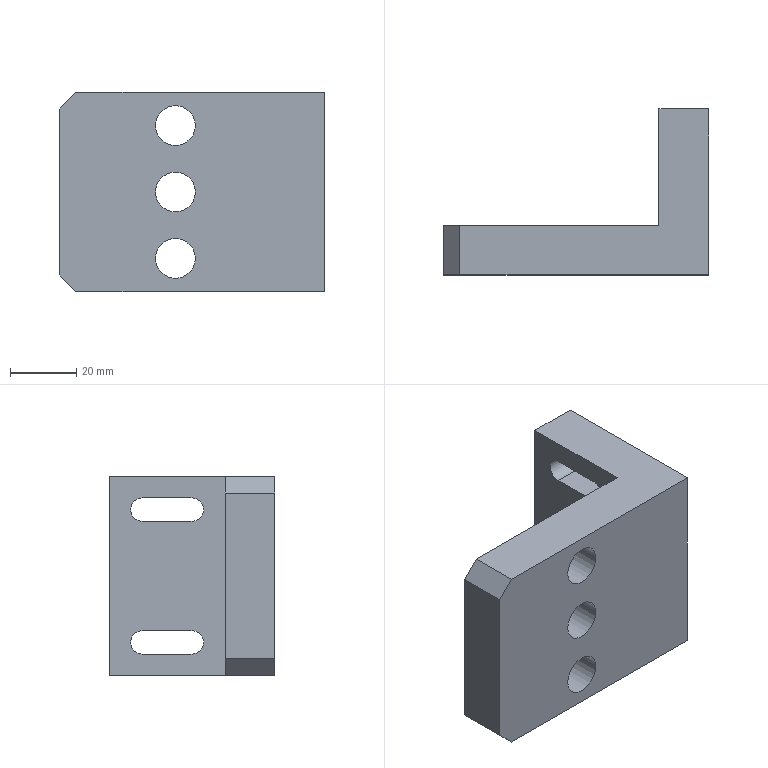Component | SolidWorks | ElectricalBoxAssembly2-1_AuxiliaryWheelAdjustmentSeat-1 | 1 solid | 24 faces | box 80 x 50 x 60 mm | volume 93731 mm3 | plane 14 | cylinder 10 | commonest cylinder face diameters 12 x6 7 x4
build123d program:
from build123d import *

# Parameters (mm, degrees)
BOSS_EXTRUDE1_DEPTH = 30
CUT_EXTRUDE1_DEPTH  = 88.321
SKETCH7_R           = 6
CUT_EXTRUDE2_DEPTH  = 93.331
CHAMFER1_SIZE       = 5


with BuildPart() as part:
    # Sketch1 → Boss-Extrude1 (new, symmetric)
    with BuildSketch(Plane.XY):
        Polygon((0, 0), (0, -50), (80, -50), (80, -35), (15, -35), (15, 0), align=None)
    extrude(amount=BOSS_EXTRUDE1_DEPTH, both=True)

    # Sketch2 → Cut-Extrude1 (cut, through all)
    with BuildSketch(Plane(origin=(15, 0, 0), x_dir=(0, 0, -1), z_dir=(1, 0, 0))):
        with BuildLine():
            Line((-16.5, -10), (-16.5, -25))
            ThreePointArc((-16.5, -25), (-20, -28.5), (-23.5, -25))
            Line((-23.5, -25), (-23.5, -10))
            ThreePointArc((-23.5, -10), (-20, -6.5), (-16.5, -10))
        make_face()
        with BuildLine():
            Line((23.5, -10), (23.5, -25))
            ThreePointArc((23.5, -25), (20, -28.5), (16.5, -25))
            Line((16.5, -25), (16.5, -10))
            ThreePointArc((16.5, -10), (20, -6.5), (23.5, -10))
        make_face()
    extrude(amount=-CUT_EXTRUDE1_DEPTH, mode=Mode.SUBTRACT)

    # Sketch7 → Cut-Extrude2 (cut, through all)
    with BuildSketch(Plane(origin=(0, -35, 0), x_dir=(1, 0, 0), z_dir=(0, 1, 0))):
        with Locations(Location((45, 20, 0), (0, 0, 180))):
            Circle(SKETCH7_R)
        with Locations(Location((45, -20, 0), (0, 0, 180))):
            Circle(SKETCH7_R)
        with Locations(Location((45, 0, 0), (0, 0, 180))):
            Circle(SKETCH7_R)
    extrude(amount=-CUT_EXTRUDE2_DEPTH, mode=Mode.SUBTRACT)

    # Chamfer1
    chamfer1_edges = [part.edges().sort_by_distance(p)[0] for p in [
        (80, -42.5, 30),
        (80, -42.5, -30),
    ]]
    chamfer(chamfer1_edges, length=CHAMFER1_SIZE)


solid = part.part

# Placed as in the assembly
solid = solid.moved(Location((755.468, 489.666, 1526.399), (-180, 0, 180)))
STEP:
#1=CARTESIAN_POINT('',(27.735,17.31,59.307));
#2=VERTEX_POINT('',#1);
#3=CARTESIAN_POINT('',(28.207,17.31,59.307));
#4=VERTEX_POINT('',#3);
#5=CARTESIAN_POINT('',(27.971,17.31,59.307));
#6=DIRECTION('',(-0.,1.,-0.));
#7=DIRECTION('',(1.,0.,0.));
#8=AXIS2_PLACEMENT_3D('',#5,#6,#7);
#9=CIRCLE('',#8,0.2362);
#10=EDGE_CURVE('',#2,#4,#9,.T.);
#11=ORIENTED_EDGE('',*,*,#10,.F.);
#12=CARTESIAN_POINT('',(27.735,17.9,59.307));
#13=VERTEX_POINT('',#12);
#14=CARTESIAN_POINT('',(27.735,17.31,59.307));
#15=DIRECTION('',(-0.,1.,-0.));
#16=VECTOR('',#15,39.37);
#17=LINE('',#14,#16);
#18=EDGE_CURVE('',#2,#13,#17,.T.);
#19=ORIENTED_EDGE('',*,*,#18,.T.);
#20=CARTESIAN_POINT('',(28.207,17.9,59.307));
#21=VERTEX_POINT('',#20);
#22=CARTESIAN_POINT('',(27.971,17.9,59.307));
#23=DIRECTION('',(-0.,1.,-0.));
#24=DIRECTION('',(1.,0.,0.));
#25=AXIS2_PLACEMENT_3D('',#22,#23,#24);
#26=CIRCLE('',#25,0.2362);
#27=EDGE_CURVE('',#13,#21,#26,.T.);
#28=ORIENTED_EDGE('',*,*,#27,.T.);
#29=CARTESIAN_POINT('',(28.207,17.31,59.307));
#30=DIRECTION('',(-0.,1.,-0.));
#31=VECTOR('',#30,39.37);
#32=LINE('',#29,#31);
#33=EDGE_CURVE('',#4,#21,#32,.T.);
#34=ORIENTED_EDGE('',*,*,#33,.F.);
#35=EDGE_LOOP('',(#11,#19,#28,#34));
#36=FACE_OUTER_BOUND('',#35,.T.);
#37=CARTESIAN_POINT('',(27.971,17.31,59.307));
#38=DIRECTION('',(-0.,1.,-0.));
#39=DIRECTION('',(1.,0.,0.));
#40=AXIS2_PLACEMENT_3D('',#37,#38,#39);
#41=CYLINDRICAL_SURFACE('',#40,0.2362);
#42=ADVANCED_FACE('',(#36),#41,.F.);
#43=CARTESIAN_POINT('',(27.735,17.31,60.094));
#44=VERTEX_POINT('',#43);
#45=CARTESIAN_POINT('',(28.207,17.31,60.094));
#46=VERTEX_POINT('',#45);
#47=CARTESIAN_POINT('',(27.971,17.31,60.094));
#48=DIRECTION('',(-0.,1.,-0.));
#49=DIRECTION('',(1.,0.,0.));
#50=AXIS2_PLACEMENT_3D('',#47,#48,#49);
#51=CIRCLE('',#50,0.2362);
#52=EDGE_CURVE('',#44,#46,#51,.T.);
#53=ORIENTED_EDGE('',*,*,#52,.F.);
#54=CARTESIAN_POINT('',(27.735,17.9,60.094));
#55=VERTEX_POINT('',#54);
#56=CARTESIAN_POINT('',(27.735,17.31,60.094));
#57=DIRECTION('',(-0.,1.,-0.));
#58=VECTOR('',#57,39.37);
#59=LINE('',#56,#58);
#60=EDGE_CURVE('',#44,#55,#59,.T.);
#61=ORIENTED_EDGE('',*,*,#60,.T.);
#62=CARTESIAN_POINT('',(28.207,17.9,60.094));
#63=VERTEX_POINT('',#62);
#64=CARTESIAN_POINT('',(27.971,17.9,60.094));
#65=DIRECTION('',(-0.,1.,-0.));
#66=DIRECTION('',(1.,0.,0.));
#67=AXIS2_PLACEMENT_3D('',#64,#65,#66);
#68=CIRCLE('',#67,0.2362);
#69=EDGE_CURVE('',#55,#63,#68,.T.);
#70=ORIENTED_EDGE('',*,*,#69,.T.);
#71=CARTESIAN_POINT('',(28.207,17.31,60.094));
#72=DIRECTION('',(-0.,1.,-0.));
#73=VECTOR('',#72,39.37);
#74=LINE('',#71,#73);
#75=EDGE_CURVE('',#46,#63,#74,.T.);
#76=ORIENTED_EDGE('',*,*,#75,.F.);
#77=EDGE_LOOP('',(#53,#61,#70,#76));
#78=FACE_OUTER_BOUND('',#77,.T.);
#79=CARTESIAN_POINT('',(27.971,17.31,60.094));
#80=DIRECTION('',(-0.,1.,-0.));
#81=DIRECTION('',(1.,0.,0.));
#82=AXIS2_PLACEMENT_3D('',#79,#80,#81);
#83=CYLINDRICAL_SURFACE('',#82,0.2362);
#84=ADVANCED_FACE('',(#78),#83,.F.);
#85=CARTESIAN_POINT('',(27.735,17.31,60.882));
#86=VERTEX_POINT('',#85);
#87=CARTESIAN_POINT('',(28.207,17.31,60.882));
#88=VERTEX_POINT('',#87);
#89=CARTESIAN_POINT('',(27.971,17.31,60.882));
#90=DIRECTION('',(-0.,1.,-0.));
#91=DIRECTION('',(1.,0.,0.));
#92=AXIS2_PLACEMENT_3D('',#89,#90,#91);
#93=CIRCLE('',#92,0.2362);
#94=EDGE_CURVE('',#86,#88,#93,.T.);
#95=ORIENTED_EDGE('',*,*,#94,.F.);
#96=CARTESIAN_POINT('',(27.735,17.9,60.882));
#97=VERTEX_POINT('',#96);
#98=CARTESIAN_POINT('',(27.735,17.31,60.882));
#99=DIRECTION('',(-0.,1.,-0.));
#100=VECTOR('',#99,39.37);
#101=LINE('',#98,#100);
#102=EDGE_CURVE('',#86,#97,#101,.T.);
#103=ORIENTED_EDGE('',*,*,#102,.T.);
#104=CARTESIAN_POINT('',(28.207,17.9,60.882));
#105=VERTEX_POINT('',#104);
#106=CARTESIAN_POINT('',(27.971,17.9,60.882));
#107=DIRECTION('',(-0.,1.,-0.));
#108=DIRECTION('',(1.,0.,0.));
#109=AXIS2_PLACEMENT_3D('',#106,#107,#108);
#110=CIRCLE('',#109,0.2362);
#111=EDGE_CURVE('',#97,#105,#110,.T.);
#112=ORIENTED_EDGE('',*,*,#111,.T.);
#113=CARTESIAN_POINT('',(28.207,17.31,60.882));
#114=DIRECTION('',(-0.,1.,-0.));
#115=VECTOR('',#114,39.37);
#116=LINE('',#113,#115);
#117=EDGE_CURVE('',#88,#105,#116,.T.);
#118=ORIENTED_EDGE('',*,*,#117,.F.);
#119=EDGE_LOOP('',(#95,#103,#112,#118));
#120=FACE_OUTER_BOUND('',#119,.T.);
#121=CARTESIAN_POINT('',(27.971,17.31,60.882));
#122=DIRECTION('',(-0.,1.,-0.));
#123=DIRECTION('',(1.,0.,0.));
#124=AXIS2_PLACEMENT_3D('',#121,#122,#123);
#125=CYLINDRICAL_SURFACE('',#124,0.2362);
#126=ADVANCED_FACE('',(#120),#125,.F.);
#127=CARTESIAN_POINT('',(29.152,19.278,61.276));
#128=VERTEX_POINT('',#127);
#129=CARTESIAN_POINT('',(29.743,19.278,61.276));
#130=VERTEX_POINT('',#129);
#131=CARTESIAN_POINT('',(29.152,19.278,61.276));
#132=DIRECTION('',(1.,0.,0.));
#133=VECTOR('',#132,39.37);
#134=LINE('',#131,#133);
#135=EDGE_CURVE('',#128,#130,#134,.T.);
#136=ORIENTED_EDGE('',*,*,#135,.T.);
#137=CARTESIAN_POINT('',(29.743,19.278,58.913));
#138=VERTEX_POINT('',#137);
#139=CARTESIAN_POINT('',(29.743,19.278,58.913));
#140=DIRECTION('',(-0.,0.,1.));
#141=VECTOR('',#140,39.37);
#142=LINE('',#139,#141);
#143=EDGE_CURVE('',#138,#130,#142,.T.);
#144=ORIENTED_EDGE('',*,*,#143,.F.);
#145=CARTESIAN_POINT('',(29.152,19.278,58.913));
#146=VERTEX_POINT('',#145);
#147=CARTESIAN_POINT('',(29.152,19.278,58.913));
#148=DIRECTION('',(1.,0.,0.));
#149=VECTOR('',#148,39.37);
#150=LINE('',#147,#149);
#151=EDGE_CURVE('',#146,#138,#150,.T.);
#152=ORIENTED_EDGE('',*,*,#151,.F.);
#153=CARTESIAN_POINT('',(29.152,19.278,58.913));
#154=DIRECTION('',(-0.,0.,1.));
#155=VECTOR('',#154,39.37);
#156=LINE('',#153,#155);
#157=EDGE_CURVE('',#146,#128,#156,.T.);
#158=ORIENTED_EDGE('',*,*,#157,.T.);
#159=EDGE_LOOP('',(#136,#144,#152,#158));
#160=FACE_OUTER_BOUND('',#159,.T.);
#161=CARTESIAN_POINT('',(29.152,19.278,58.913));
#162=DIRECTION('',(0.,-1.,0.));
#163=DIRECTION('',(-1.,-0.,-0.));
#164=AXIS2_PLACEMENT_3D('',#161,#162,#163);
#165=PLANE('',#164);
#166=ADVANCED_FACE('',(#160),#165,.F.);
#167=CARTESIAN_POINT('',(29.743,18.294,61.02));
#168=VERTEX_POINT('',#167);
#169=CARTESIAN_POINT('',(29.743,18.884,61.02));
#170=VERTEX_POINT('',#169);
#171=CARTESIAN_POINT('',(29.743,18.884,61.02));
#172=DIRECTION('',(-0.,1.,-0.));
#173=VECTOR('',#172,39.37);
#174=LINE('',#171,#173);
#175=EDGE_CURVE('',#168,#170,#174,.T.);
#176=ORIENTED_EDGE('',*,*,#175,.T.);
#177=CARTESIAN_POINT('',(29.743,18.884,60.744));
#178=VERTEX_POINT('',#177);
#179=CARTESIAN_POINT('',(29.743,18.884,60.882));
#180=DIRECTION('',(-1.,-0.,-0.));
#181=DIRECTION('',(0.,0.,1.));
#182=AXIS2_PLACEMENT_3D('',#179,#180,#181);
#183=CIRCLE('',#182,0.1378);
#184=EDGE_CURVE('',#170,#178,#183,.T.);
#185=ORIENTED_EDGE('',*,*,#184,.T.);
#186=CARTESIAN_POINT('',(29.743,18.294,60.744));
#187=VERTEX_POINT('',#186);
#188=CARTESIAN_POINT('',(29.743,18.884,60.744));
#189=DIRECTION('',(0.,-1.,0.));
#190=VECTOR('',#189,39.37);
#191=LINE('',#188,#190);
#192=EDGE_CURVE('',#178,#187,#191,.T.);
#193=ORIENTED_EDGE('',*,*,#192,.T.);
#194=CARTESIAN_POINT('',(29.743,18.294,60.882));
#195=DIRECTION('',(-1.,-0.,-0.));
#196=DIRECTION('',(0.,0.,1.));
#197=AXIS2_PLACEMENT_3D('',#194,#195,#196);
#198=CIRCLE('',#197,0.1378);
#199=EDGE_CURVE('',#187,#168,#198,.T.);
#200=ORIENTED_EDGE('',*,*,#199,.T.);
#201=EDGE_LOOP('',(#176,#185,#193,#200));
#202=FACE_BOUND('',#201,.T.);
#203=CARTESIAN_POINT('',(29.743,18.294,59.445));
#204=VERTEX_POINT('',#203);
#205=CARTESIAN_POINT('',(29.743,18.884,59.445));
#206=VERTEX_POINT('',#205);
#207=CARTESIAN_POINT('',(29.743,18.884,59.445));
#208=DIRECTION('',(-0.,1.,-0.));
#209=VECTOR('',#208,39.37);
#210=LINE('',#207,#209);
#211=EDGE_CURVE('',#204,#206,#210,.T.);
#212=ORIENTED_EDGE('',*,*,#211,.T.);
#213=CARTESIAN_POINT('',(29.743,18.884,59.169));
#214=VERTEX_POINT('',#213);
#215=CARTESIAN_POINT('',(29.743,18.884,59.307));
#216=DIRECTION('',(-1.,-0.,-0.));
#217=DIRECTION('',(0.,0.,1.));
#218=AXIS2_PLACEMENT_3D('',#215,#216,#217);
#219=CIRCLE('',#218,0.1378);
#220=EDGE_CURVE('',#206,#214,#219,.T.);
#221=ORIENTED_EDGE('',*,*,#220,.T.);
#222=CARTESIAN_POINT('',(29.743,18.294,59.169));
#223=VERTEX_POINT('',#222);
#224=CARTESIAN_POINT('',(29.743,18.884,59.169));
#225=DIRECTION('',(0.,-1.,0.));
#226=VECTOR('',#225,39.37);
#227=LINE('',#224,#226);
#228=EDGE_CURVE('',#214,#223,#227,.T.);
#229=ORIENTED_EDGE('',*,*,#228,.T.);
#230=CARTESIAN_POINT('',(29.743,18.294,59.307));
#231=DIRECTION('',(-1.,-0.,-0.));
#232=DIRECTION('',(0.,0.,1.));
#233=AXIS2_PLACEMENT_3D('',#230,#231,#232);
#234=CIRCLE('',#233,0.1378);
#235=EDGE_CURVE('',#223,#204,#234,.T.);
#236=ORIENTED_EDGE('',*,*,#235,.T.);
#237=EDGE_LOOP('',(#212,#221,#229,#236));
#238=FACE_BOUND('',#237,.T.);
#239=CARTESIAN_POINT('',(29.743,17.31,61.276));
#240=VERTEX_POINT('',#239);
#241=CARTESIAN_POINT('',(29.743,19.278,61.276));
#242=DIRECTION('',(0.,-1.,0.));
#243=VECTOR('',#242,39.37);
#244=LINE('',#241,#243);
#245=EDGE_CURVE('',#130,#240,#244,.T.);
#246=ORIENTED_EDGE('',*,*,#245,.T.);
#247=CARTESIAN_POINT('',(29.743,17.31,58.913));
#248=VERTEX_POINT('',#247);
#249=CARTESIAN_POINT('',(29.743,17.31,58.913));
#250=DIRECTION('',(-0.,0.,1.));
#251=VECTOR('',#250,39.37);
#252=LINE('',#249,#251);
#253=EDGE_CURVE('',#248,#240,#252,.T.);
#254=ORIENTED_EDGE('',*,*,#253,.F.);
#255=CARTESIAN_POINT('',(29.743,19.278,58.913));
#256=DIRECTION('',(0.,-1.,0.));
#257=VECTOR('',#256,39.37);
#258=LINE('',#255,#257);
#259=EDGE_CURVE('',#138,#248,#258,.T.);
#260=ORIENTED_EDGE('',*,*,#259,.F.);
#261=ORIENTED_EDGE('',*,*,#143,.T.);
#262=EDGE_LOOP('',(#246,#254,#260,#261));
#263=FACE_OUTER_BOUND('',#262,.T.);
#264=CARTESIAN_POINT('',(29.743,19.278,58.913));
#265=DIRECTION('',(-1.,-0.,-0.));
#266=DIRECTION('',(-0.,1.,-0.));
#267=AXIS2_PLACEMENT_3D('',#264,#265,#266);
#268=PLANE('',#267);
#269=ADVANCED_FACE('',(#202,#238,#263),#268,.F.);
#270=CARTESIAN_POINT('',(27.971,17.31,59.307));
#271=DIRECTION('',(-0.,1.,-0.));
#272=DIRECTION('',(1.,0.,0.));
#273=AXIS2_PLACEMENT_3D('',#270,#271,#272);
#274=CIRCLE('',#273,0.2362);
#275=EDGE_CURVE('',#4,#2,#274,.T.);
#276=ORIENTED_EDGE('',*,*,#275,.T.);
#277=ORIENTED_EDGE('',*,*,#10,.T.);
#278=EDGE_LOOP('',(#276,#277));
#279=FACE_BOUND('',#278,.T.);
#280=CARTESIAN_POINT('',(27.971,17.31,60.094));
#281=DIRECTION('',(-0.,1.,-0.));
#282=DIRECTION('',(1.,0.,0.));
#283=AXIS2_PLACEMENT_3D('',#280,#281,#282);
#284=CIRCLE('',#283,0.2362);
#285=EDGE_CURVE('',#46,#44,#284,.T.);
#286=ORIENTED_EDGE('',*,*,#285,.T.);
#287=ORIENTED_EDGE('',*,*,#52,.T.);
#288=EDGE_LOOP('',(#286,#287));
#289=FACE_BOUND('',#288,.T.);
#290=CARTESIAN_POINT('',(27.971,17.31,60.882));
#291=DIRECTION('',(-0.,1.,-0.));
#292=DIRECTION('',(1.,0.,0.));
#293=AXIS2_PLACEMENT_3D('',#290,#291,#292);
#294=CIRCLE('',#293,0.2362);
#295=EDGE_CURVE('',#88,#86,#294,.T.);
#296=ORIENTED_EDGE('',*,*,#295,.T.);
#297=ORIENTED_EDGE('',*,*,#94,.T.);
#298=EDGE_LOOP('',(#296,#297));
#299=FACE_BOUND('',#298,.T.);
#300=CARTESIAN_POINT('',(26.593,17.31,59.11));
#301=VERTEX_POINT('',#300);
#302=CARTESIAN_POINT('',(26.593,17.31,61.079));
#303=VERTEX_POINT('',#302);
#304=CARTESIAN_POINT('',(26.593,17.31,58.913));
#305=DIRECTION('',(-0.,0.,1.));
#306=VECTOR('',#305,39.37);
#307=LINE('',#304,#306);
#308=EDGE_CURVE('',#301,#303,#307,.T.);
#309=ORIENTED_EDGE('',*,*,#308,.F.);
#310=CARTESIAN_POINT('',(26.79,17.31,58.913));
#311=VERTEX_POINT('',#310);
#312=CARTESIAN_POINT('',(26.79,17.31,58.913));
#313=DIRECTION('',(0.7071,0.,-0.7071));
#314=VECTOR('',#313,39.37);
#315=LINE('',#312,#314);
#316=EDGE_CURVE('',#301,#311,#315,.T.);
#317=ORIENTED_EDGE('',*,*,#316,.T.);
#318=CARTESIAN_POINT('',(29.743,17.31,58.913));
#319=DIRECTION('',(-1.,-0.,-0.));
#320=VECTOR('',#319,39.37);
#321=LINE('',#318,#320);
#322=EDGE_CURVE('',#248,#311,#321,.T.);
#323=ORIENTED_EDGE('',*,*,#322,.F.);
#324=ORIENTED_EDGE('',*,*,#253,.T.);
#325=CARTESIAN_POINT('',(26.79,17.31,61.276));
#326=VERTEX_POINT('',#325);
#327=CARTESIAN_POINT('',(29.743,17.31,61.276));
#328=DIRECTION('',(-1.,-0.,-0.));
#329=VECTOR('',#328,39.37);
#330=LINE('',#327,#329);
#331=EDGE_CURVE('',#240,#326,#330,.T.);
#332=ORIENTED_EDGE('',*,*,#331,.T.);
#333=CARTESIAN_POINT('',(26.593,17.31,61.079));
#334=DIRECTION('',(-0.7071,-0.,-0.7071));
#335=VECTOR('',#334,39.37);
#336=LINE('',#333,#335);
#337=EDGE_CURVE('',#326,#303,#336,.T.);
#338=ORIENTED_EDGE('',*,*,#337,.T.);
#339=EDGE_LOOP('',(#309,#317,#323,#324,#332,#338));
#340=FACE_OUTER_BOUND('',#339,.T.);
#341=CARTESIAN_POINT('',(29.743,17.31,58.913));
#342=DIRECTION('',(-0.,1.,-0.));
#343=DIRECTION('',(0.,-0.,-1.));
#344=AXIS2_PLACEMENT_3D('',#341,#342,#343);
#345=PLANE('',#344);
#346=ADVANCED_FACE('',(#279,#289,#299,#340),#345,.F.);
#347=CARTESIAN_POINT('',(26.593,17.9,59.11));
#348=VERTEX_POINT('',#347);
#349=CARTESIAN_POINT('',(26.593,17.9,61.079));
#350=VERTEX_POINT('',#349);
#351=CARTESIAN_POINT('',(26.593,17.9,58.913));
#352=DIRECTION('',(-0.,0.,1.));
#353=VECTOR('',#352,39.37);
#354=LINE('',#351,#353);
#355=EDGE_CURVE('',#348,#350,#354,.T.);
#356=ORIENTED_EDGE('',*,*,#355,.F.);
#357=CARTESIAN_POINT('',(26.593,17.31,59.11));
#358=DIRECTION('',(0.,-1.,0.));
#359=VECTOR('',#358,39.37);
#360=LINE('',#357,#359);
#361=EDGE_CURVE('',#348,#301,#360,.T.);
#362=ORIENTED_EDGE('',*,*,#361,.T.);
#363=ORIENTED_EDGE('',*,*,#308,.T.);
#364=CARTESIAN_POINT('',(26.593,17.31,61.079));
#365=DIRECTION('',(-0.,1.,-0.));
#366=VECTOR('',#365,39.37);
#367=LINE('',#364,#366);
#368=EDGE_CURVE('',#303,#350,#367,.T.);
#369=ORIENTED_EDGE('',*,*,#368,.T.);
#370=EDGE_LOOP('',(#356,#362,#363,#369));
#371=FACE_OUTER_BOUND('',#370,.T.);
#372=CARTESIAN_POINT('',(26.593,17.31,58.913));
#373=DIRECTION('',(1.,0.,0.));
#374=DIRECTION('',(0.,-0.,-1.));
#375=AXIS2_PLACEMENT_3D('',#372,#373,#374);
#376=PLANE('',#375);
#377=ADVANCED_FACE('',(#371),#376,.F.);
#378=CARTESIAN_POINT('',(27.971,17.9,59.307));
#379=DIRECTION('',(-0.,1.,-0.));
#380=DIRECTION('',(1.,0.,0.));
#381=AXIS2_PLACEMENT_3D('',#378,#379,#380);
#382=CIRCLE('',#381,0.2362);
#383=EDGE_CURVE('',#21,#13,#382,.T.);
#384=ORIENTED_EDGE('',*,*,#383,.F.);
#385=ORIENTED_EDGE('',*,*,#27,.F.);
#386=EDGE_LOOP('',(#384,#385));
#387=FACE_BOUND('',#386,.T.);
#388=CARTESIAN_POINT('',(27.971,17.9,60.094));
#389=DIRECTION('',(-0.,1.,-0.));
#390=DIRECTION('',(1.,0.,0.));
#391=AXIS2_PLACEMENT_3D('',#388,#389,#390);
#392=CIRCLE('',#391,0.2362);
#393=EDGE_CURVE('',#63,#55,#392,.T.);
#394=ORIENTED_EDGE('',*,*,#393,.F.);
#395=ORIENTED_EDGE('',*,*,#69,.F.);
#396=EDGE_LOOP('',(#394,#395));
#397=FACE_BOUND('',#396,.T.);
#398=CARTESIAN_POINT('',(27.971,17.9,60.882));
#399=DIRECTION('',(-0.,1.,-0.));
#400=DIRECTION('',(1.,0.,0.));
#401=AXIS2_PLACEMENT_3D('',#398,#399,#400);
#402=CIRCLE('',#401,0.2362);
#403=EDGE_CURVE('',#105,#97,#402,.T.);
#404=ORIENTED_EDGE('',*,*,#403,.F.);
#405=ORIENTED_EDGE('',*,*,#111,.F.);
#406=EDGE_LOOP('',(#404,#405));
#407=FACE_BOUND('',#406,.T.);
#408=CARTESIAN_POINT('',(26.79,17.9,58.913));
#409=VERTEX_POINT('',#408);
#410=CARTESIAN_POINT('',(29.152,17.9,58.913));
#411=VERTEX_POINT('',#410);
#412=CARTESIAN_POINT('',(26.593,17.9,58.913));
#413=DIRECTION('',(1.,0.,0.));
#414=VECTOR('',#413,39.37);
#415=LINE('',#412,#414);
#416=EDGE_CURVE('',#409,#411,#415,.T.);
#417=ORIENTED_EDGE('',*,*,#416,.F.);
#418=CARTESIAN_POINT('',(26.79,17.9,58.913));
#419=DIRECTION('',(-0.7071,-0.,0.7071));
#420=VECTOR('',#419,39.37);
#421=LINE('',#418,#420);
#422=EDGE_CURVE('',#409,#348,#421,.T.);
#423=ORIENTED_EDGE('',*,*,#422,.T.);
#424=ORIENTED_EDGE('',*,*,#355,.T.);
#425=CARTESIAN_POINT('',(26.79,17.9,61.276));
#426=VERTEX_POINT('',#425);
#427=CARTESIAN_POINT('',(26.593,17.9,61.079));
#428=DIRECTION('',(0.7071,0.,0.7071));
#429=VECTOR('',#428,39.37);
#430=LINE('',#427,#429);
#431=EDGE_CURVE('',#350,#426,#430,.T.);
#432=ORIENTED_EDGE('',*,*,#431,.T.);
#433=CARTESIAN_POINT('',(29.152,17.9,61.276));
#434=VERTEX_POINT('',#433);
#435=CARTESIAN_POINT('',(26.593,17.9,61.276));
#436=DIRECTION('',(1.,0.,0.));
#437=VECTOR('',#436,39.37);
#438=LINE('',#435,#437);
#439=EDGE_CURVE('',#426,#434,#438,.T.);
#440=ORIENTED_EDGE('',*,*,#439,.T.);
#441=CARTESIAN_POINT('',(29.152,17.9,58.913));
#442=DIRECTION('',(-0.,0.,1.));
#443=VECTOR('',#442,39.37);
#444=LINE('',#441,#443);
#445=EDGE_CURVE('',#411,#434,#444,.T.);
#446=ORIENTED_EDGE('',*,*,#445,.F.);
#447=EDGE_LOOP('',(#417,#423,#424,#432,#440,#446));
#448=FACE_OUTER_BOUND('',#447,.T.);
#449=CARTESIAN_POINT('',(26.593,17.9,58.913));
#450=DIRECTION('',(0.,-1.,0.));
#451=DIRECTION('',(-1.,-0.,-0.));
#452=AXIS2_PLACEMENT_3D('',#449,#450,#451);
#453=PLANE('',#452);
#454=ADVANCED_FACE('',(#387,#397,#407,#448),#453,.F.);
#455=CARTESIAN_POINT('',(29.152,18.884,60.744));
#456=VERTEX_POINT('',#455);
#457=CARTESIAN_POINT('',(29.152,18.294,60.744));
#458=VERTEX_POINT('',#457);
#459=CARTESIAN_POINT('',(29.152,18.884,60.744));
#460=DIRECTION('',(0.,-1.,0.));
#461=VECTOR('',#460,39.37);
#462=LINE('',#459,#461);
#463=EDGE_CURVE('',#456,#458,#462,.T.);
#464=ORIENTED_EDGE('',*,*,#463,.F.);
#465=CARTESIAN_POINT('',(29.152,18.884,61.02));
#466=VERTEX_POINT('',#465);
#467=CARTESIAN_POINT('',(29.152,18.884,60.882));
#468=DIRECTION('',(-1.,-0.,-0.));
#469=DIRECTION('',(0.,0.,1.));
#470=AXIS2_PLACEMENT_3D('',#467,#468,#469);
#471=CIRCLE('',#470,0.1378);
#472=EDGE_CURVE('',#466,#456,#471,.T.);
#473=ORIENTED_EDGE('',*,*,#472,.F.);
#474=CARTESIAN_POINT('',(29.152,18.294,61.02));
#475=VERTEX_POINT('',#474);
#476=CARTESIAN_POINT('',(29.152,18.884,61.02));
#477=DIRECTION('',(-0.,1.,-0.));
#478=VECTOR('',#477,39.37);
#479=LINE('',#476,#478);
#480=EDGE_CURVE('',#475,#466,#479,.T.);
#481=ORIENTED_EDGE('',*,*,#480,.F.);
#482=CARTESIAN_POINT('',(29.152,18.294,60.882));
#483=DIRECTION('',(-1.,-0.,-0.));
#484=DIRECTION('',(0.,0.,1.));
#485=AXIS2_PLACEMENT_3D('',#482,#483,#484);
#486=CIRCLE('',#485,0.1378);
#487=EDGE_CURVE('',#458,#475,#486,.T.);
#488=ORIENTED_EDGE('',*,*,#487,.F.);
#489=EDGE_LOOP('',(#464,#473,#481,#488));
#490=FACE_BOUND('',#489,.T.);
#491=CARTESIAN_POINT('',(29.152,18.884,59.169));
#492=VERTEX_POINT('',#491);
#493=CARTESIAN_POINT('',(29.152,18.294,59.169));
#494=VERTEX_POINT('',#493);
#495=CARTESIAN_POINT('',(29.152,18.884,59.169));
#496=DIRECTION('',(0.,-1.,0.));
#497=VECTOR('',#496,39.37);
#498=LINE('',#495,#497);
#499=EDGE_CURVE('',#492,#494,#498,.T.);
#500=ORIENTED_EDGE('',*,*,#499,.F.);
#501=CARTESIAN_POINT('',(29.152,18.884,59.445));
#502=VERTEX_POINT('',#501);
#503=CARTESIAN_POINT('',(29.152,18.884,59.307));
#504=DIRECTION('',(-1.,-0.,-0.));
#505=DIRECTION('',(0.,0.,1.));
#506=AXIS2_PLACEMENT_3D('',#503,#504,#505);
#507=CIRCLE('',#506,0.1378);
#508=EDGE_CURVE('',#502,#492,#507,.T.);
#509=ORIENTED_EDGE('',*,*,#508,.F.);
#510=CARTESIAN_POINT('',(29.152,18.294,59.445));
#511=VERTEX_POINT('',#510);
#512=CARTESIAN_POINT('',(29.152,18.884,59.445));
#513=DIRECTION('',(-0.,1.,-0.));
#514=VECTOR('',#513,39.37);
#515=LINE('',#512,#514);
#516=EDGE_CURVE('',#511,#502,#515,.T.);
#517=ORIENTED_EDGE('',*,*,#516,.F.);
#518=CARTESIAN_POINT('',(29.152,18.294,59.307));
#519=DIRECTION('',(-1.,-0.,-0.));
#520=DIRECTION('',(0.,0.,1.));
#521=AXIS2_PLACEMENT_3D('',#518,#519,#520);
#522=CIRCLE('',#521,0.1378);
#523=EDGE_CURVE('',#494,#511,#522,.T.);
#524=ORIENTED_EDGE('',*,*,#523,.F.);
#525=EDGE_LOOP('',(#500,#509,#517,#524));
#526=FACE_BOUND('',#525,.T.);
#527=CARTESIAN_POINT('',(29.152,17.9,61.276));
#528=DIRECTION('',(-0.,1.,-0.));
#529=VECTOR('',#528,39.37);
#530=LINE('',#527,#529);
#531=EDGE_CURVE('',#434,#128,#530,.T.);
#532=ORIENTED_EDGE('',*,*,#531,.T.);
#533=ORIENTED_EDGE('',*,*,#157,.F.);
#534=CARTESIAN_POINT('',(29.152,17.9,58.913));
#535=DIRECTION('',(-0.,1.,-0.));
#536=VECTOR('',#535,39.37);
#537=LINE('',#534,#536);
#538=EDGE_CURVE('',#411,#146,#537,.T.);
#539=ORIENTED_EDGE('',*,*,#538,.F.);
#540=ORIENTED_EDGE('',*,*,#445,.T.);
#541=EDGE_LOOP('',(#532,#533,#539,#540));
#542=FACE_OUTER_BOUND('',#541,.T.);
#543=CARTESIAN_POINT('',(29.152,17.9,58.913));
#544=DIRECTION('',(1.,0.,0.));
#545=DIRECTION('',(0.,-0.,-1.));
#546=AXIS2_PLACEMENT_3D('',#543,#544,#545);
#547=PLANE('',#546);
#548=ADVANCED_FACE('',(#490,#526,#542),#547,.F.);
#549=ORIENTED_EDGE('',*,*,#322,.T.);
#550=CARTESIAN_POINT('',(26.79,17.9,58.913));
#551=DIRECTION('',(-0.,1.,-0.));
#552=VECTOR('',#551,39.37);
#553=LINE('',#550,#552);
#554=EDGE_CURVE('',#311,#409,#553,.T.);
#555=ORIENTED_EDGE('',*,*,#554,.T.);
#556=ORIENTED_EDGE('',*,*,#416,.T.);
#557=ORIENTED_EDGE('',*,*,#538,.T.);
#558=ORIENTED_EDGE('',*,*,#151,.T.);
#559=ORIENTED_EDGE('',*,*,#259,.T.);
#560=EDGE_LOOP('',(#549,#555,#556,#557,#558,#559));
#561=FACE_OUTER_BOUND('',#560,.T.);
#562=CARTESIAN_POINT('',(29.743,19.278,58.913));
#563=DIRECTION('',(0.,-0.,-1.));
#564=DIRECTION('',(-1.,-0.,-0.));
#565=AXIS2_PLACEMENT_3D('',#562,#563,#564);
#566=PLANE('',#565);
#567=ADVANCED_FACE('',(#561),#566,.T.);
#568=ORIENTED_EDGE('',*,*,#439,.F.);
#569=CARTESIAN_POINT('',(26.79,19.278,61.276));
#570=DIRECTION('',(0.,-1.,0.));
#571=VECTOR('',#570,39.37);
#572=LINE('',#569,#571);
#573=EDGE_CURVE('',#426,#326,#572,.T.);
#574=ORIENTED_EDGE('',*,*,#573,.T.);
#575=ORIENTED_EDGE('',*,*,#331,.F.);
#576=ORIENTED_EDGE('',*,*,#245,.F.);
#577=ORIENTED_EDGE('',*,*,#135,.F.);
#578=ORIENTED_EDGE('',*,*,#531,.F.);
#579=EDGE_LOOP('',(#568,#574,#575,#576,#577,#578));
#580=FACE_OUTER_BOUND('',#579,.T.);
#581=CARTESIAN_POINT('',(29.743,19.278,61.276));
#582=DIRECTION('',(0.,-0.,-1.));
#583=DIRECTION('',(-1.,-0.,-0.));
#584=AXIS2_PLACEMENT_3D('',#581,#582,#583);
#585=PLANE('',#584);
#586=ADVANCED_FACE('',(#580),#585,.F.);
#587=ORIENTED_EDGE('',*,*,#508,.T.);
#588=CARTESIAN_POINT('',(29.743,18.884,59.169));
#589=DIRECTION('',(-1.,-0.,-0.));
#590=VECTOR('',#589,39.37);
#591=LINE('',#588,#590);
#592=EDGE_CURVE('',#214,#492,#591,.T.);
#593=ORIENTED_EDGE('',*,*,#592,.F.);
#594=ORIENTED_EDGE('',*,*,#220,.F.);
#595=CARTESIAN_POINT('',(29.743,18.884,59.445));
#596=DIRECTION('',(-1.,-0.,-0.));
#597=VECTOR('',#596,39.37);
#598=LINE('',#595,#597);
#599=EDGE_CURVE('',#206,#502,#598,.T.);
#600=ORIENTED_EDGE('',*,*,#599,.T.);
#601=EDGE_LOOP('',(#587,#593,#594,#600));
#602=FACE_OUTER_BOUND('',#601,.T.);
#603=CARTESIAN_POINT('',(29.743,18.884,59.307));
#604=DIRECTION('',(-1.,-0.,-0.));
#605=DIRECTION('',(0.,0.,1.));
#606=AXIS2_PLACEMENT_3D('',#603,#604,#605);
#607=CYLINDRICAL_SURFACE('',#606,0.1378);
#608=ADVANCED_FACE('',(#602),#607,.F.);
#609=ORIENTED_EDGE('',*,*,#516,.T.);
#610=ORIENTED_EDGE('',*,*,#599,.F.);
#611=ORIENTED_EDGE('',*,*,#211,.F.);
#612=CARTESIAN_POINT('',(29.743,18.294,59.445));
#613=DIRECTION('',(-1.,-0.,-0.));
#614=VECTOR('',#613,39.37);
#615=LINE('',#612,#614);
#616=EDGE_CURVE('',#204,#511,#615,.T.);
#617=ORIENTED_EDGE('',*,*,#616,.T.);
#618=EDGE_LOOP('',(#609,#610,#611,#617));
#619=FACE_OUTER_BOUND('',#618,.T.);
#620=CARTESIAN_POINT('',(29.743,18.884,59.445));
#621=DIRECTION('',(-0.,0.,1.));
#622=DIRECTION('',(1.,0.,0.));
#623=AXIS2_PLACEMENT_3D('',#620,#621,#622);
#624=PLANE('',#623);
#625=ADVANCED_FACE('',(#619),#624,.F.);
#626=ORIENTED_EDGE('',*,*,#523,.T.);
#627=ORIENTED_EDGE('',*,*,#616,.F.);
#628=ORIENTED_EDGE('',*,*,#235,.F.);
#629=CARTESIAN_POINT('',(29.743,18.294,59.169));
#630=DIRECTION('',(-1.,-0.,-0.));
#631=VECTOR('',#630,39.37);
#632=LINE('',#629,#631);
#633=EDGE_CURVE('',#223,#494,#632,.T.);
#634=ORIENTED_EDGE('',*,*,#633,.T.);
#635=EDGE_LOOP('',(#626,#627,#628,#634));
#636=FACE_OUTER_BOUND('',#635,.T.);
#637=CARTESIAN_POINT('',(29.743,18.294,59.307));
#638=DIRECTION('',(-1.,-0.,-0.));
#639=DIRECTION('',(0.,0.,1.));
#640=AXIS2_PLACEMENT_3D('',#637,#638,#639);
#641=CYLINDRICAL_SURFACE('',#640,0.1378);
#642=ADVANCED_FACE('',(#636),#641,.F.);
#643=ORIENTED_EDGE('',*,*,#499,.T.);
#644=ORIENTED_EDGE('',*,*,#633,.F.);
#645=ORIENTED_EDGE('',*,*,#228,.F.);
#646=ORIENTED_EDGE('',*,*,#592,.T.);
#647=EDGE_LOOP('',(#643,#644,#645,#646));
#648=FACE_OUTER_BOUND('',#647,.T.);
#649=CARTESIAN_POINT('',(29.743,18.884,59.169));
#650=DIRECTION('',(0.,-0.,-1.));
#651=DIRECTION('',(-1.,-0.,-0.));
#652=AXIS2_PLACEMENT_3D('',#649,#650,#651);
#653=PLANE('',#652);
#654=ADVANCED_FACE('',(#648),#653,.F.);
#655=ORIENTED_EDGE('',*,*,#472,.T.);
#656=CARTESIAN_POINT('',(29.743,18.884,60.744));
#657=DIRECTION('',(-1.,-0.,-0.));
#658=VECTOR('',#657,39.37);
#659=LINE('',#656,#658);
#660=EDGE_CURVE('',#178,#456,#659,.T.);
#661=ORIENTED_EDGE('',*,*,#660,.F.);
#662=ORIENTED_EDGE('',*,*,#184,.F.);
#663=CARTESIAN_POINT('',(29.743,18.884,61.02));
#664=DIRECTION('',(-1.,-0.,-0.));
#665=VECTOR('',#664,39.37);
#666=LINE('',#663,#665);
#667=EDGE_CURVE('',#170,#466,#666,.T.);
#668=ORIENTED_EDGE('',*,*,#667,.T.);
#669=EDGE_LOOP('',(#655,#661,#662,#668));
#670=FACE_OUTER_BOUND('',#669,.T.);
#671=CARTESIAN_POINT('',(29.743,18.884,60.882));
#672=DIRECTION('',(-1.,-0.,-0.));
#673=DIRECTION('',(0.,0.,1.));
#674=AXIS2_PLACEMENT_3D('',#671,#672,#673);
#675=CYLINDRICAL_SURFACE('',#674,0.1378);
#676=ADVANCED_FACE('',(#670),#675,.F.);
#677=ORIENTED_EDGE('',*,*,#480,.T.);
#678=ORIENTED_EDGE('',*,*,#667,.F.);
#679=ORIENTED_EDGE('',*,*,#175,.F.);
#680=CARTESIAN_POINT('',(29.743,18.294,61.02));
#681=DIRECTION('',(-1.,-0.,-0.));
#682=VECTOR('',#681,39.37);
#683=LINE('',#680,#682);
#684=EDGE_CURVE('',#168,#475,#683,.T.);
#685=ORIENTED_EDGE('',*,*,#684,.T.);
#686=EDGE_LOOP('',(#677,#678,#679,#685));
#687=FACE_OUTER_BOUND('',#686,.T.);
#688=CARTESIAN_POINT('',(29.743,18.884,61.02));
#689=DIRECTION('',(-0.,0.,1.));
#690=DIRECTION('',(1.,0.,0.));
#691=AXIS2_PLACEMENT_3D('',#688,#689,#690);
#692=PLANE('',#691);
#693=ADVANCED_FACE('',(#687),#692,.F.);
#694=ORIENTED_EDGE('',*,*,#487,.T.);
#695=ORIENTED_EDGE('',*,*,#684,.F.);
#696=ORIENTED_EDGE('',*,*,#199,.F.);
#697=CARTESIAN_POINT('',(29.743,18.294,60.744));
#698=DIRECTION('',(-1.,-0.,-0.));
#699=VECTOR('',#698,39.37);
#700=LINE('',#697,#699);
#701=EDGE_CURVE('',#187,#458,#700,.T.);
#702=ORIENTED_EDGE('',*,*,#701,.T.);
#703=EDGE_LOOP('',(#694,#695,#696,#702));
#704=FACE_OUTER_BOUND('',#703,.T.);
#705=CARTESIAN_POINT('',(29.743,18.294,60.882));
#706=DIRECTION('',(-1.,-0.,-0.));
#707=DIRECTION('',(0.,0.,1.));
#708=AXIS2_PLACEMENT_3D('',#705,#706,#707);
#709=CYLINDRICAL_SURFACE('',#708,0.1378);
#710=ADVANCED_FACE('',(#704),#709,.F.);
#711=ORIENTED_EDGE('',*,*,#463,.T.);
#712=ORIENTED_EDGE('',*,*,#701,.F.);
#713=ORIENTED_EDGE('',*,*,#192,.F.);
#714=ORIENTED_EDGE('',*,*,#660,.T.);
#715=EDGE_LOOP('',(#711,#712,#713,#714));
#716=FACE_OUTER_BOUND('',#715,.T.);
#717=CARTESIAN_POINT('',(29.743,18.884,60.744));
#718=DIRECTION('',(0.,-0.,-1.));
#719=DIRECTION('',(-1.,-0.,-0.));
#720=AXIS2_PLACEMENT_3D('',#717,#718,#719);
#721=PLANE('',#720);
#722=ADVANCED_FACE('',(#716),#721,.F.);
#723=ORIENTED_EDGE('',*,*,#102,.F.);
#724=ORIENTED_EDGE('',*,*,#295,.F.);
#725=ORIENTED_EDGE('',*,*,#117,.T.);
#726=ORIENTED_EDGE('',*,*,#403,.T.);
#727=EDGE_LOOP('',(#723,#724,#725,#726));
#728=FACE_OUTER_BOUND('',#727,.T.);
#729=CARTESIAN_POINT('',(27.971,17.31,60.882));
#730=DIRECTION('',(-0.,1.,-0.));
#731=DIRECTION('',(1.,0.,0.));
#732=AXIS2_PLACEMENT_3D('',#729,#730,#731);
#733=CYLINDRICAL_SURFACE('',#732,0.2362);
#734=ADVANCED_FACE('',(#728),#733,.F.);
#735=ORIENTED_EDGE('',*,*,#60,.F.);
#736=ORIENTED_EDGE('',*,*,#285,.F.);
#737=ORIENTED_EDGE('',*,*,#75,.T.);
#738=ORIENTED_EDGE('',*,*,#393,.T.);
#739=EDGE_LOOP('',(#735,#736,#737,#738));
#740=FACE_OUTER_BOUND('',#739,.T.);
#741=CARTESIAN_POINT('',(27.971,17.31,60.094));
#742=DIRECTION('',(-0.,1.,-0.));
#743=DIRECTION('',(1.,0.,0.));
#744=AXIS2_PLACEMENT_3D('',#741,#742,#743);
#745=CYLINDRICAL_SURFACE('',#744,0.2362);
#746=ADVANCED_FACE('',(#740),#745,.F.);
#747=ORIENTED_EDGE('',*,*,#18,.F.);
#748=ORIENTED_EDGE('',*,*,#275,.F.);
#749=ORIENTED_EDGE('',*,*,#33,.T.);
#750=ORIENTED_EDGE('',*,*,#383,.T.);
#751=EDGE_LOOP('',(#747,#748,#749,#750));
#752=FACE_OUTER_BOUND('',#751,.T.);
#753=CARTESIAN_POINT('',(27.971,17.31,59.307));
#754=DIRECTION('',(-0.,1.,-0.));
#755=DIRECTION('',(1.,0.,0.));
#756=AXIS2_PLACEMENT_3D('',#753,#754,#755);
#757=CYLINDRICAL_SURFACE('',#756,0.2362);
#758=ADVANCED_FACE('',(#752),#757,.F.);
#759=ORIENTED_EDGE('',*,*,#316,.F.);
#760=ORIENTED_EDGE('',*,*,#361,.F.);
#761=ORIENTED_EDGE('',*,*,#422,.F.);
#762=ORIENTED_EDGE('',*,*,#554,.F.);
#763=EDGE_LOOP('',(#759,#760,#761,#762));
#764=FACE_OUTER_BOUND('',#763,.T.);
#765=CARTESIAN_POINT('',(26.79,19.278,58.913));
#766=DIRECTION('',(-0.7071,-0.,-0.7071));
#767=DIRECTION('',(0.,-1.,0.));
#768=AXIS2_PLACEMENT_3D('',#765,#766,#767);
#769=PLANE('',#768);
#770=ADVANCED_FACE('',(#764),#769,.T.);
#771=ORIENTED_EDGE('',*,*,#337,.F.);
#772=ORIENTED_EDGE('',*,*,#573,.F.);
#773=ORIENTED_EDGE('',*,*,#431,.F.);
#774=ORIENTED_EDGE('',*,*,#368,.F.);
#775=EDGE_LOOP('',(#771,#772,#773,#774));
#776=FACE_OUTER_BOUND('',#775,.T.);
#777=CARTESIAN_POINT('',(26.593,17.31,61.079));
#778=DIRECTION('',(0.7071,0.,-0.7071));
#779=DIRECTION('',(-0.,1.,-0.));
#780=AXIS2_PLACEMENT_3D('',#777,#778,#779);
#781=PLANE('',#780);
#782=ADVANCED_FACE('',(#776),#781,.F.);
#783=CLOSED_SHELL('',(#42,#84,#126,#166,#269,#346,#377,#454,#548,#567,#586,#608,#625,#642,#654,#676,#693,#710,#722,#734,#746,#758,#770,#782));
#784=MANIFOLD_SOLID_BREP('',#783);
#785=CARTESIAN_POINT('',(0.,0.,0.));
#786=DIRECTION('',(0.,0.,1.));
#787=DIRECTION('',(1.,0.,0.));
#788=AXIS2_PLACEMENT_3D('',#785,#786,#787);
#789=(LENGTH_UNIT()NAMED_UNIT(*)SI_UNIT($,.METRE.));
#790=LENGTH_MEASURE_WITH_UNIT(LENGTH_MEASURE(0.0254),#789);
#791=DIMENSIONAL_EXPONENTS(1.,0.,0.,0.,0.,0.,0.);
#792=(CONVERSION_BASED_UNIT('',#790)LENGTH_UNIT()NAMED_UNIT(#791));
#793=UNCERTAINTY_MEASURE_WITH_UNIT(LENGTH_MEASURE(0.00001),#792,'','');
#794=(NAMED_UNIT(*)PLANE_ANGLE_UNIT()SI_UNIT($,.RADIAN.));
#795=(NAMED_UNIT(*)SI_UNIT($,.STERADIAN.)SOLID_ANGLE_UNIT());
#796=(GEOMETRIC_REPRESENTATION_CONTEXT(3)GLOBAL_UNCERTAINTY_ASSIGNED_CONTEXT((#793))GLOBAL_UNIT_ASSIGNED_CONTEXT((#792,#794,#795))REPRESENTATION_CONTEXT('',''));
#797=ADVANCED_BREP_SHAPE_REPRESENTATION('',(#784,#788),#796);
#798=COLOUR_RGB('',0.7922,0.8196,0.9333);
#799=FILL_AREA_STYLE_COLOUR('',#798);
#800=FILL_AREA_STYLE('',(#799));
#801=SURFACE_STYLE_FILL_AREA(#800);
#802=SURFACE_SIDE_STYLE('',(#801));
#803=SURFACE_STYLE_USAGE(.BOTH.,#802);
#804=PRESENTATION_STYLE_ASSIGNMENT((#803));
#805=STYLED_ITEM('',(#804),#784);
#806=(LENGTH_UNIT()NAMED_UNIT(*)SI_UNIT($,.METRE.));
#807=LENGTH_MEASURE_WITH_UNIT(LENGTH_MEASURE(0.0254),#806);
#808=DIMENSIONAL_EXPONENTS(1.,0.,0.,0.,0.,0.,0.);
#809=(CONVERSION_BASED_UNIT('',#807)LENGTH_UNIT()NAMED_UNIT(#808));
#810=UNCERTAINTY_MEASURE_WITH_UNIT(LENGTH_MEASURE(0.00001),#809,'','');
#811=(NAMED_UNIT(*)PLANE_ANGLE_UNIT()SI_UNIT($,.RADIAN.));
#812=(NAMED_UNIT(*)SI_UNIT($,.STERADIAN.)SOLID_ANGLE_UNIT());
#813=(GEOMETRIC_REPRESENTATION_CONTEXT(3)GLOBAL_UNCERTAINTY_ASSIGNED_CONTEXT((#810))GLOBAL_UNIT_ASSIGNED_CONTEXT((#809,#811,#812))REPRESENTATION_CONTEXT('',''));
#814=MECHANICAL_DESIGN_GEOMETRIC_PRESENTATION_REPRESENTATION('',(#805),#813);
#815=PRESENTATION_LAYER_ASSIGNMENT('','',(#805));